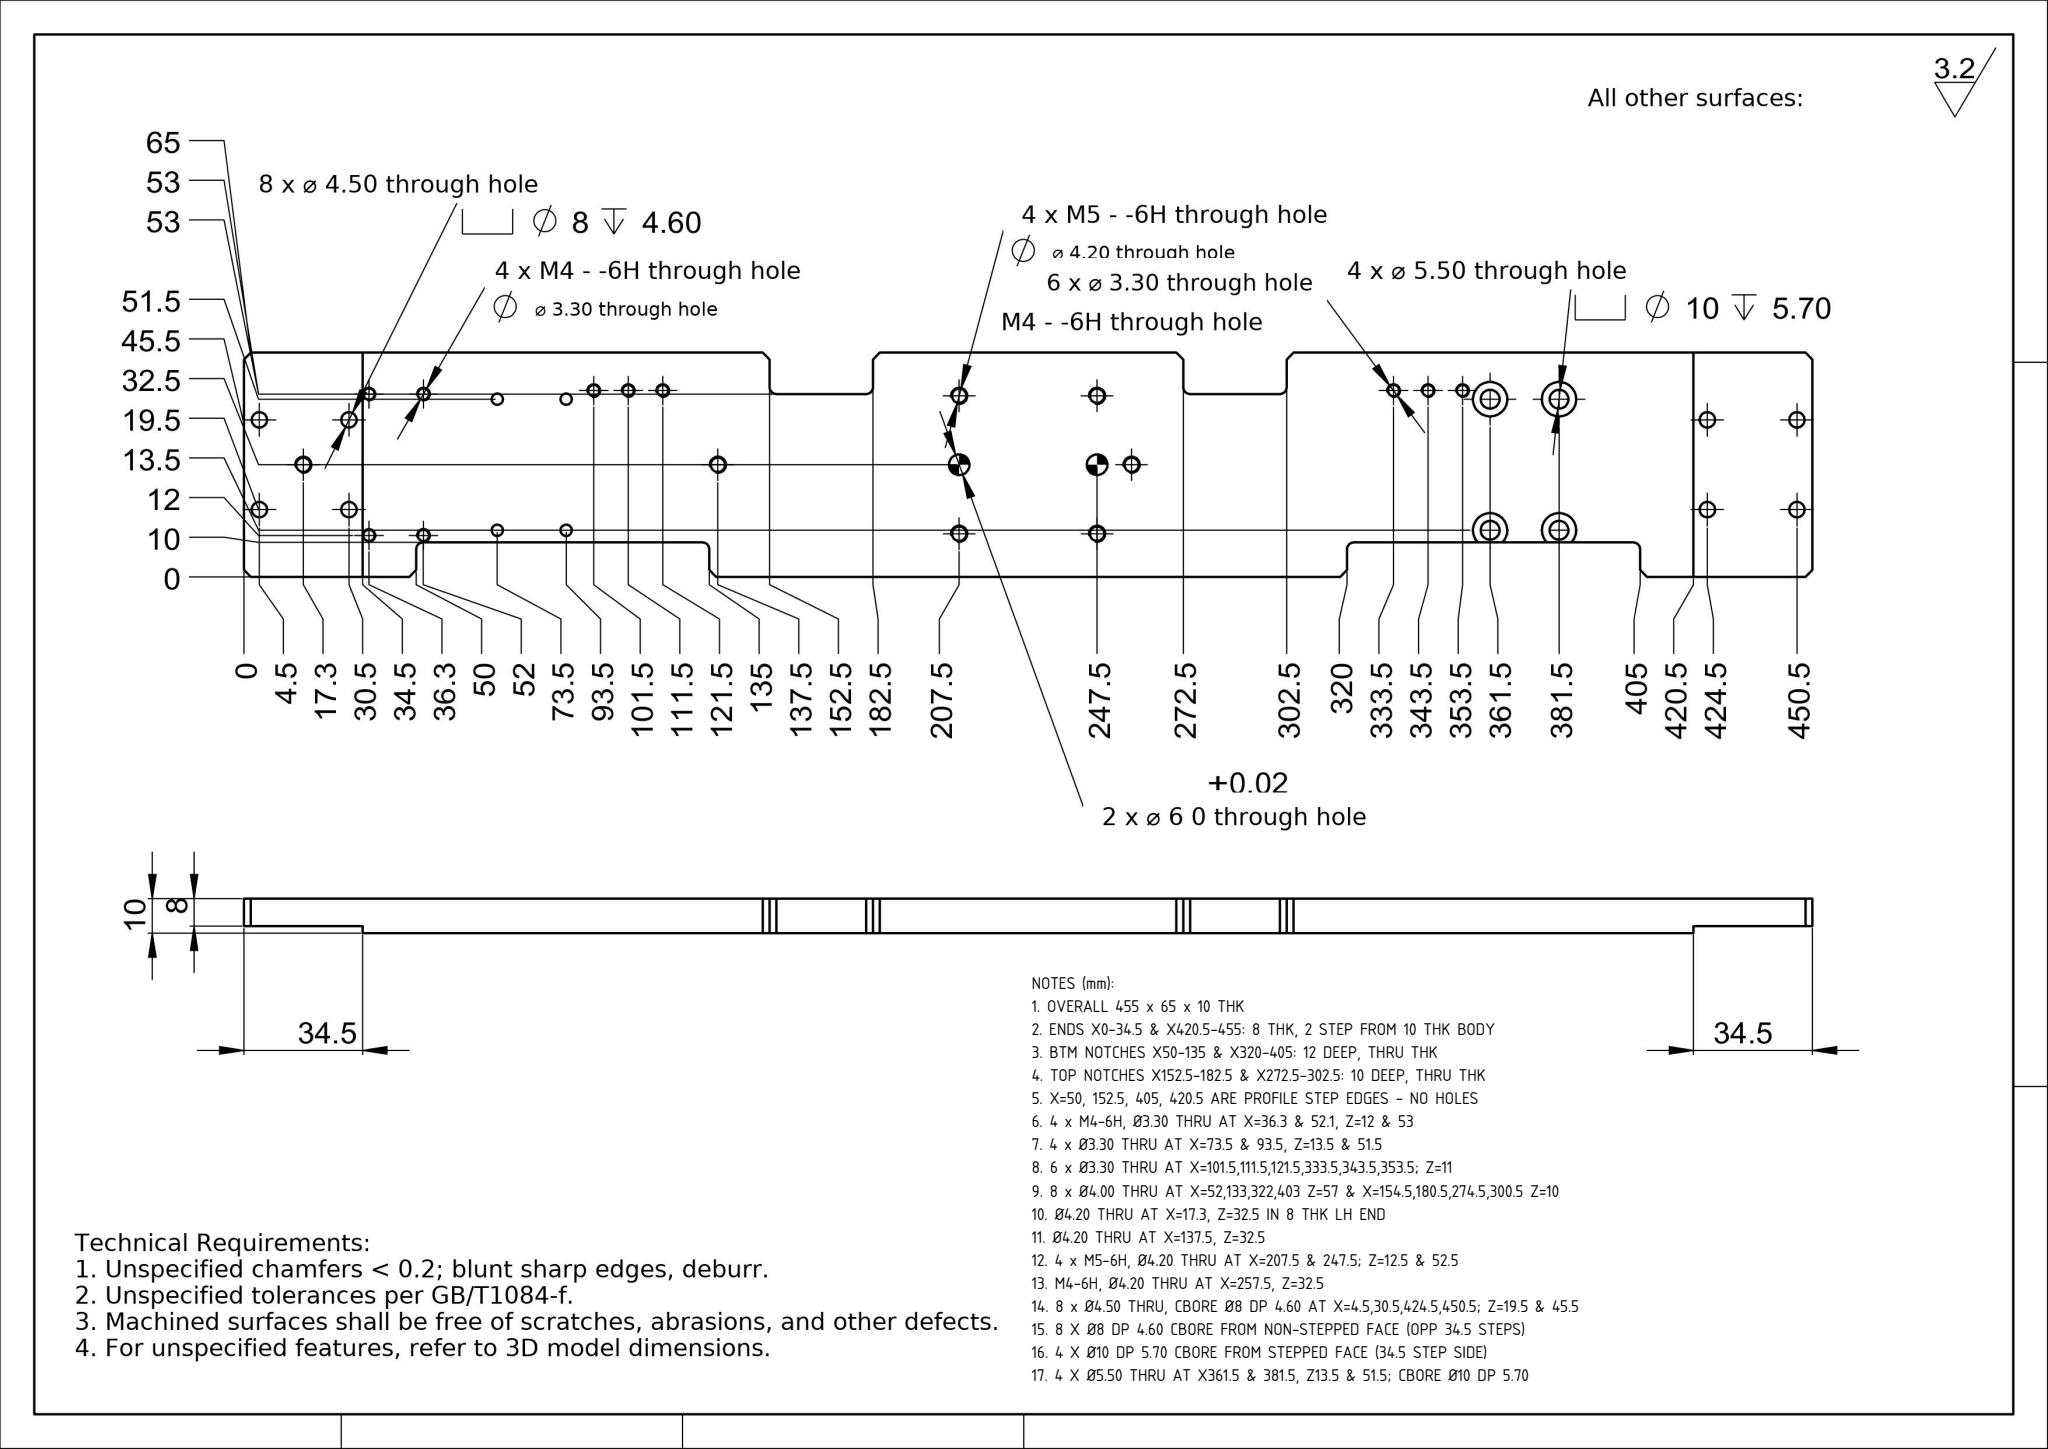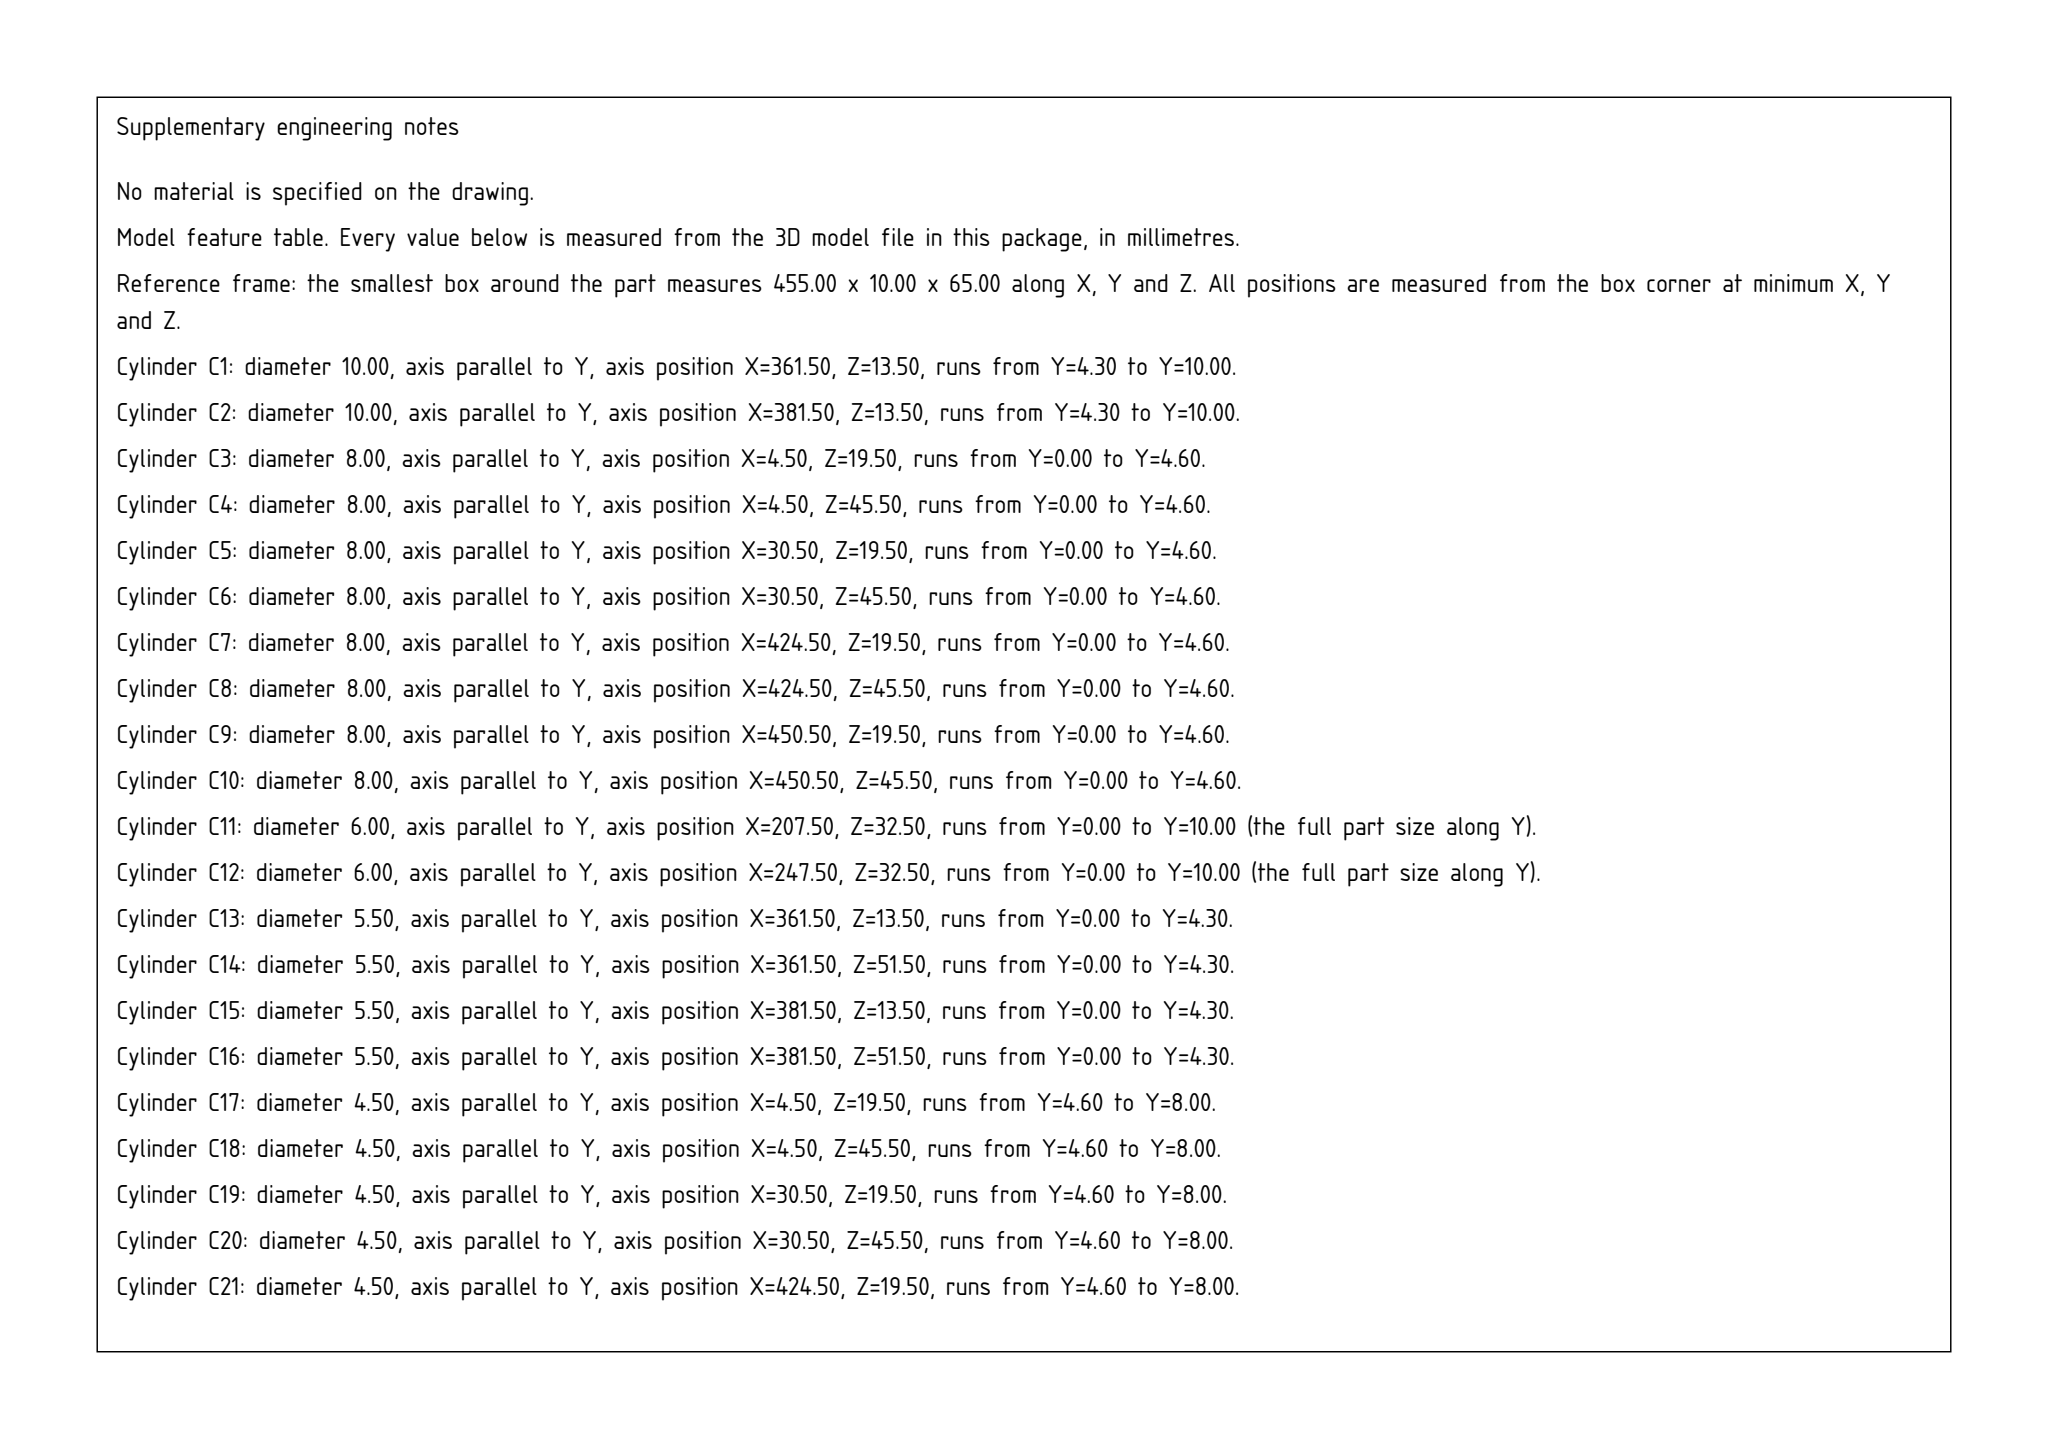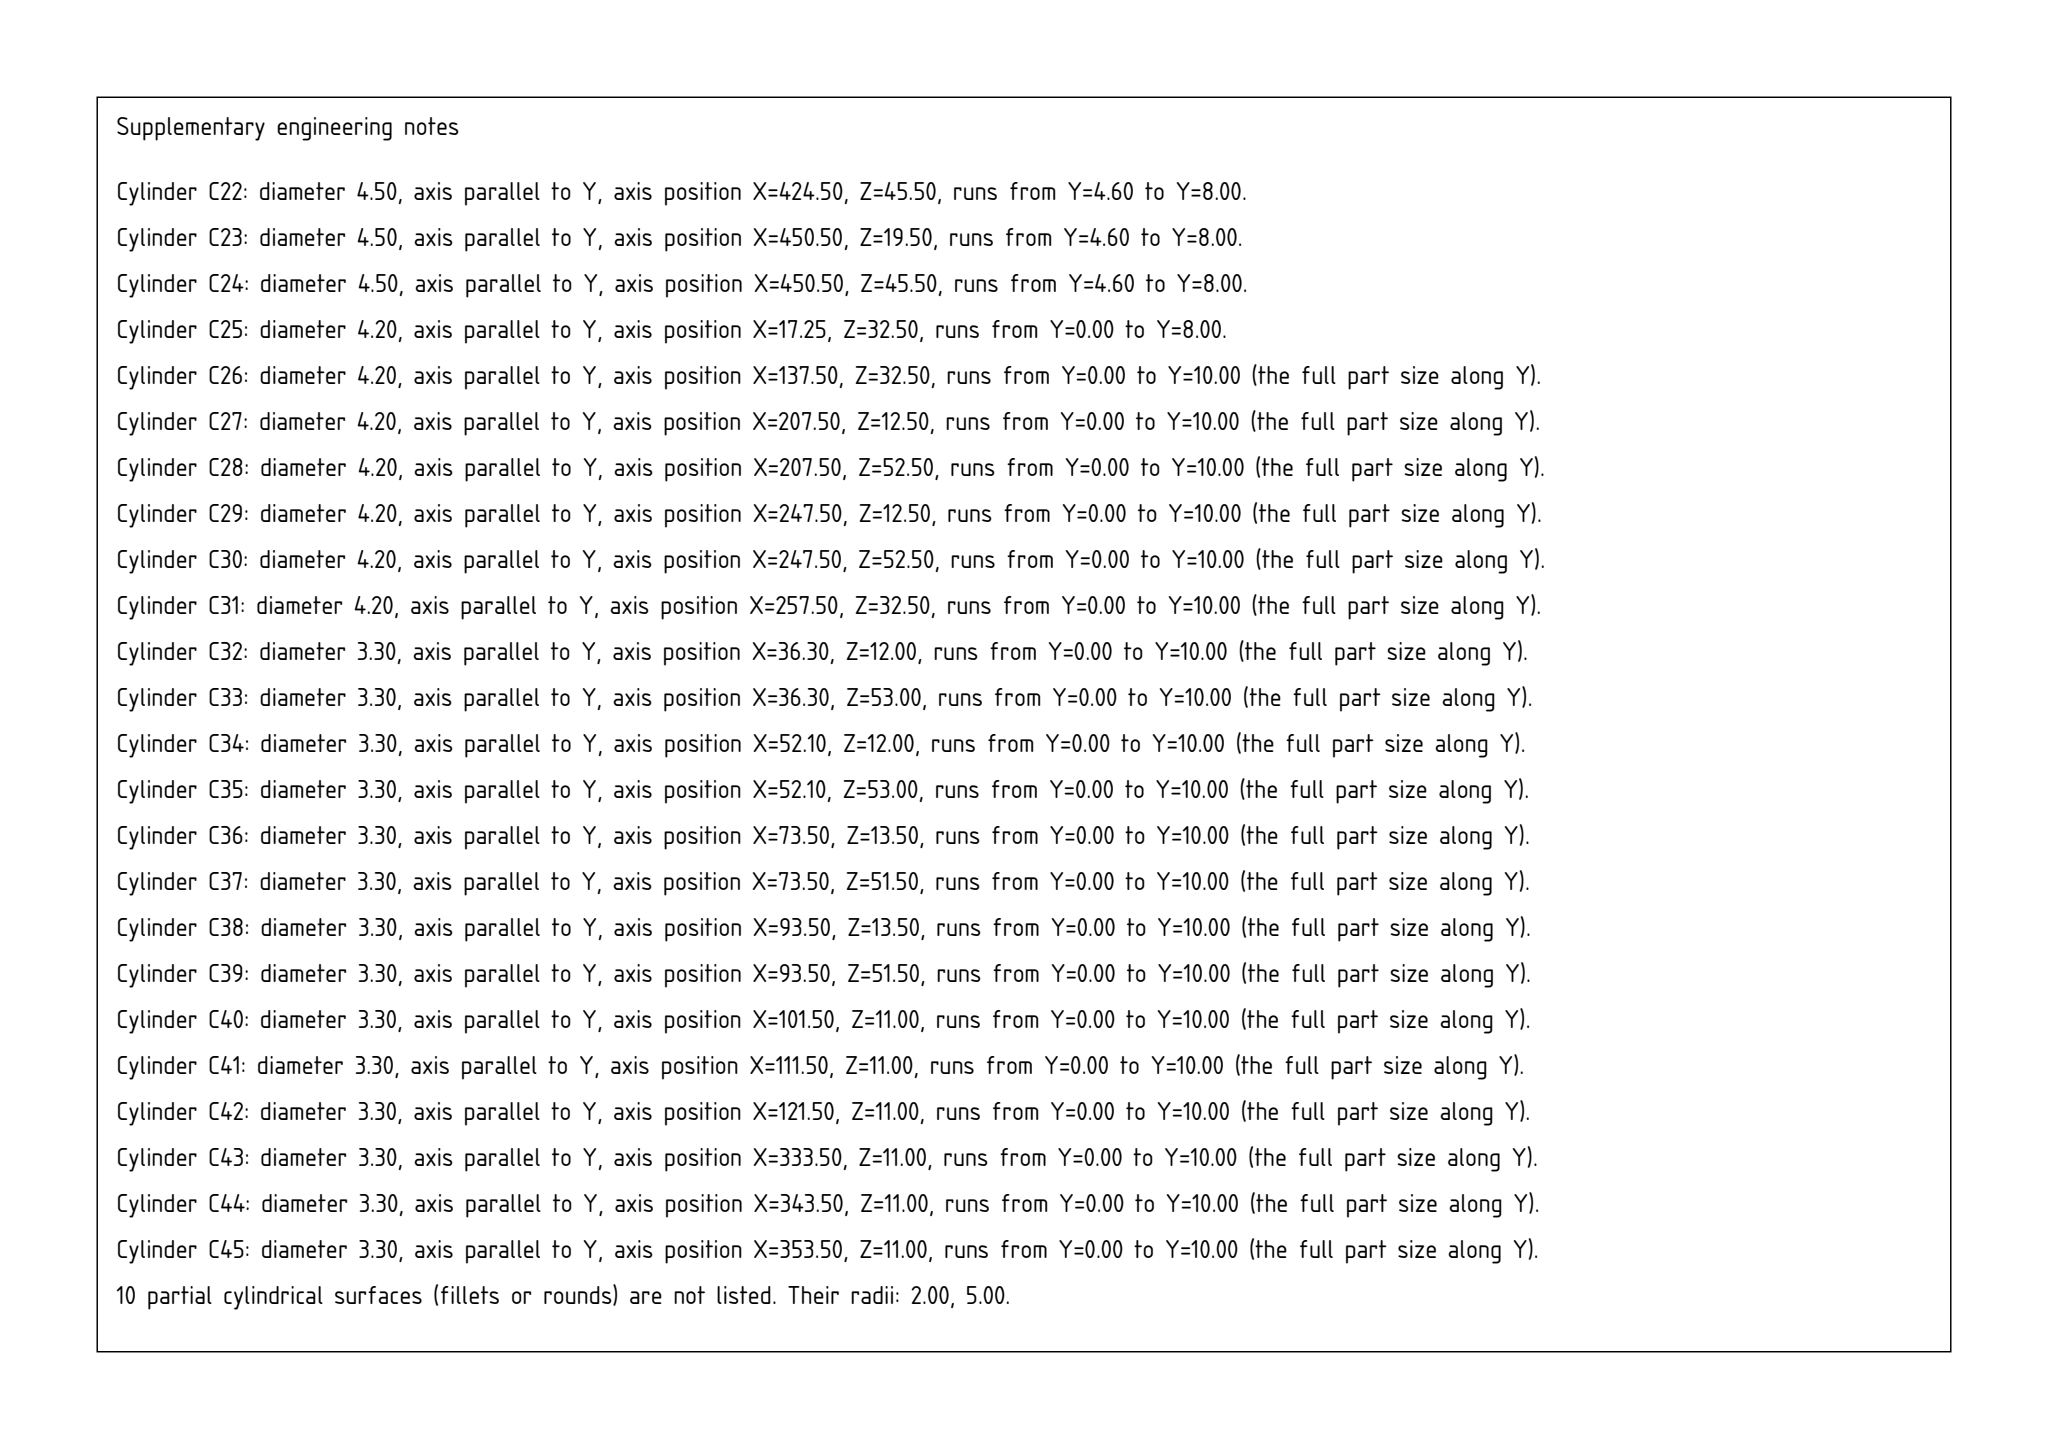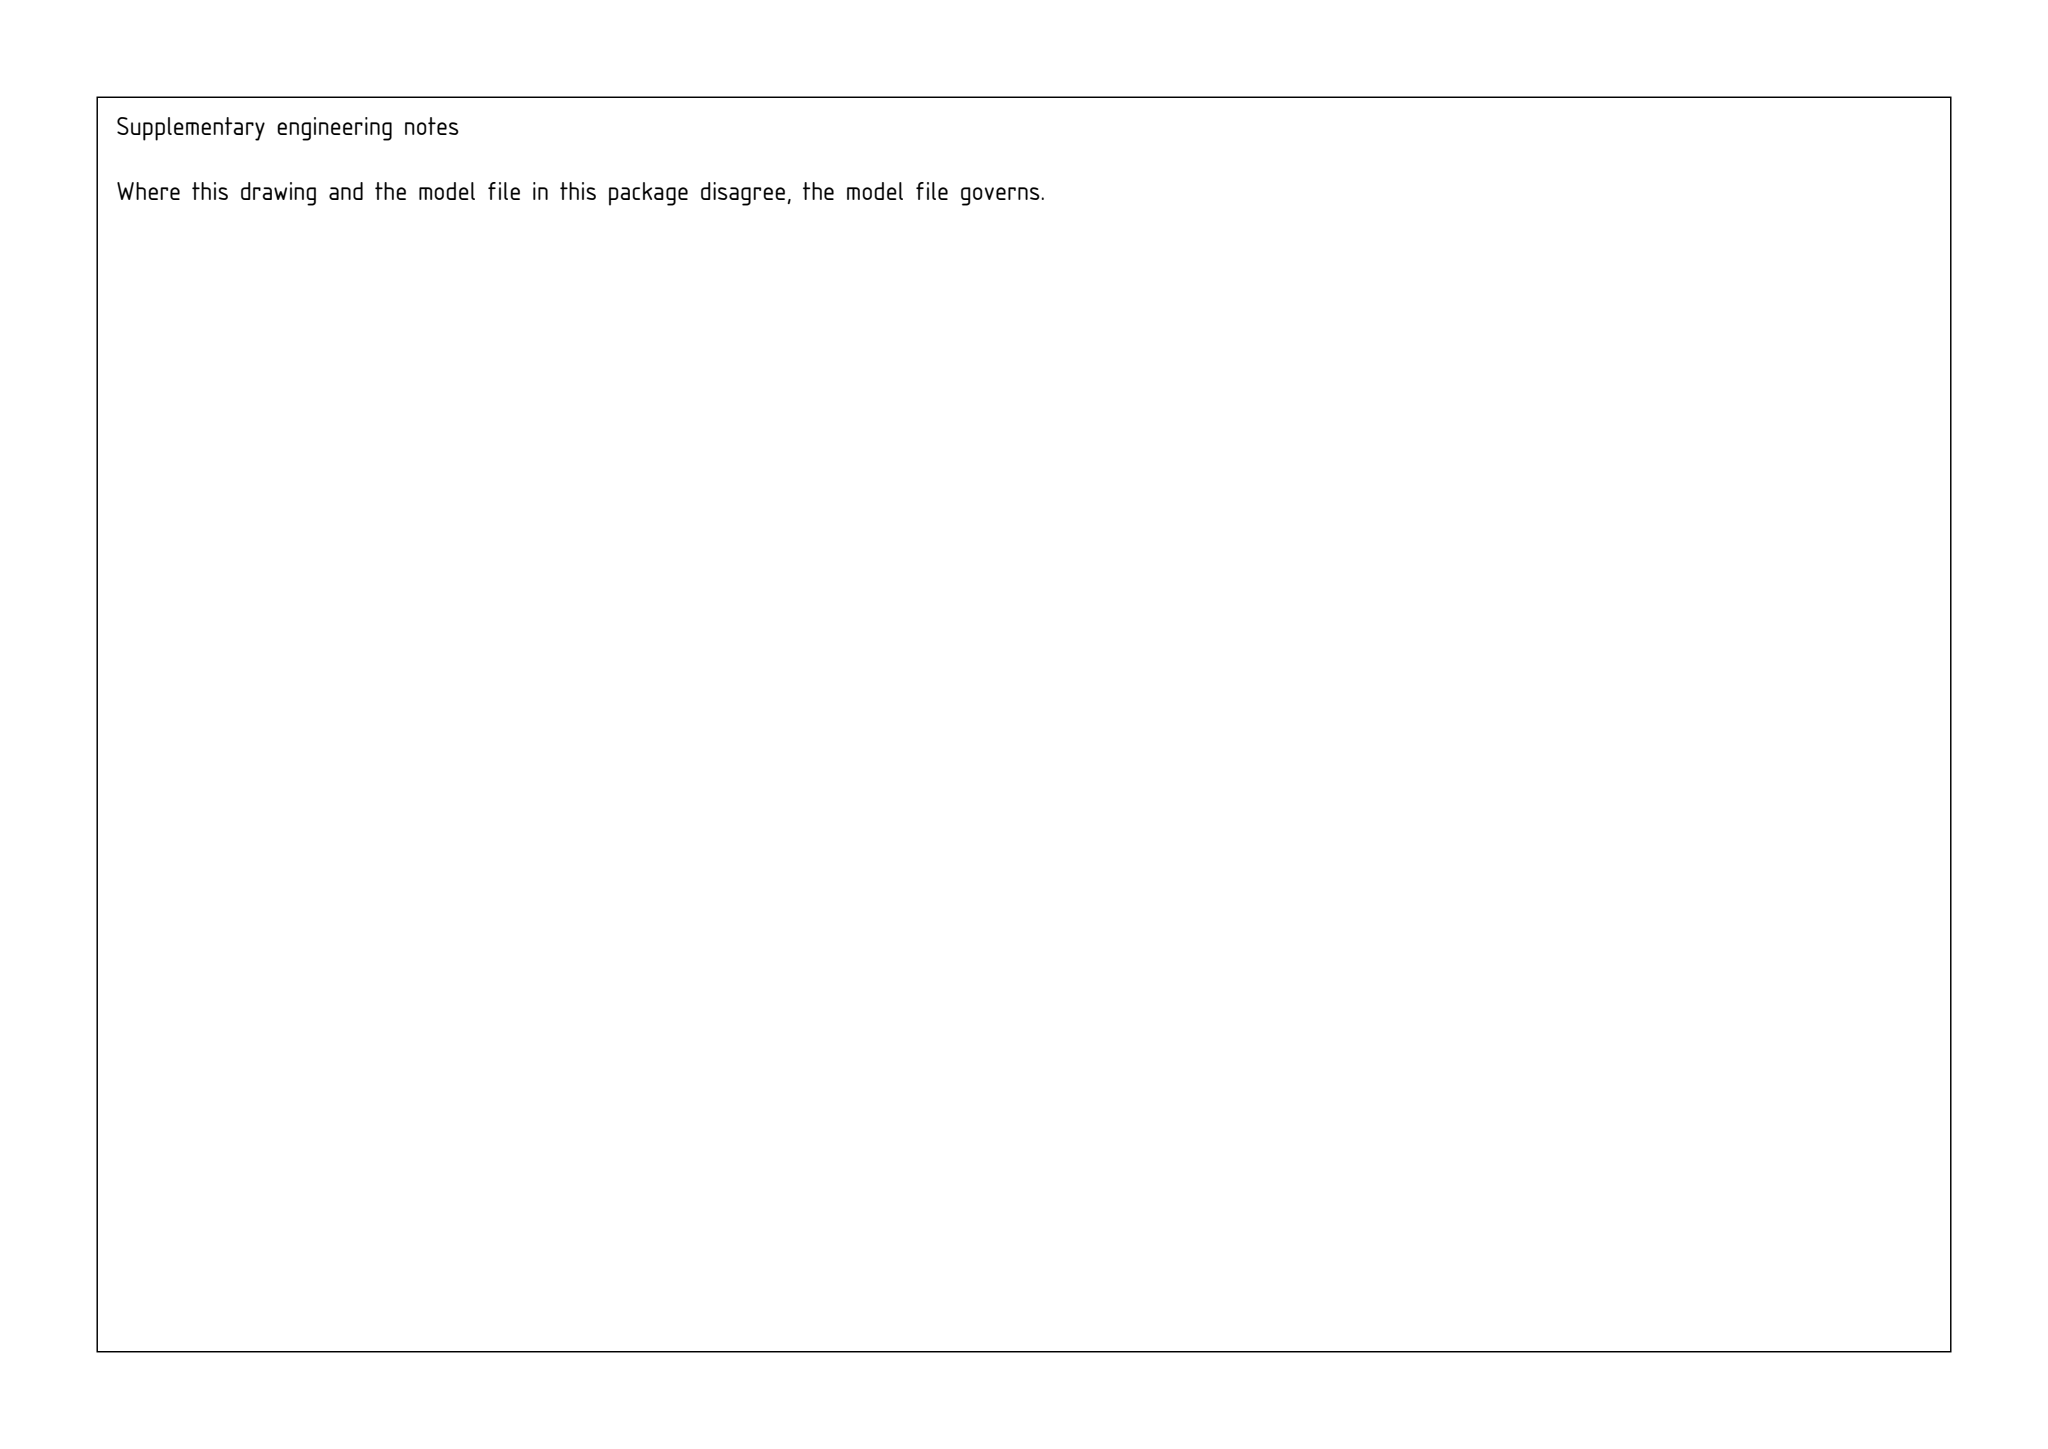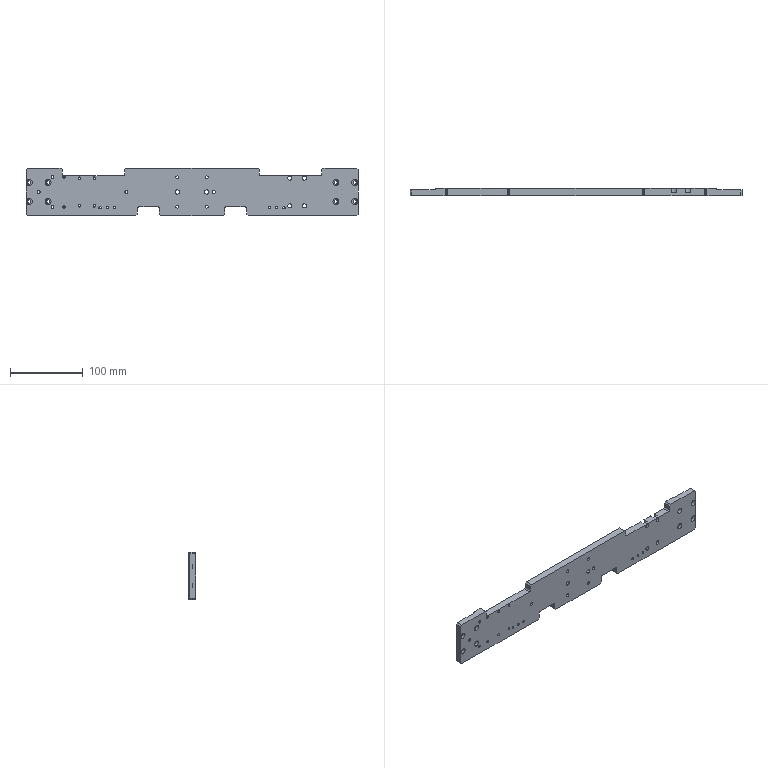Part | SolidWorks | mm | 1 solid | 150 faces | box 455 x 10 x 65 mm | volume 255322 mm3 | cylinder 100 | plane 50 | commonest cylinder face diameters 3.3 x28 8 x16 4.5 x16 4.2 x14 5.5 x8 4 x8 10 x6 6 x4
Drawing notes:
OVERALL 455 x 65 x 10 THK | from the solid: bbox_xyz 455.0 x 10.0 x 65.0
ENDS X0-34.5 & X420.5-455: 8 THK, 2 STEP FROM 10 THK BODY | from the solid: y planes 0, 8(2), 10(1); bbox y=10
BTM NOTCHES X50-135 & X320-405: 12 DEEP, THRU THK | from the solid: z planes 0(3) and 12(2); x planes 50,135,320,405
TOP NOTCHES X152.5-182.5 & X272.5-302.5: 10 DEEP, THRU THK | from the solid: z planes 65(3) and 55(2); x planes 152.5,182.5,272.5,302.5
X=50, 152.5, 405, 420.5 ARE PROFILE STEP EDGES - NO HOLES | from the solid: axis_planes x at 50,152.5,405,420.5; no cylinders at these x
4 x M4-6H, Ø3.30 THRU AT X=36.3 & 52.1, Z=12 & 53 | from the solid: cyl dia3.3 axis y at (36.3,12),(36.3,53),(52.1,12),(52.1,53), len 10
4 x Ø3.30 THRU AT X=73.5 & 93.5, Z=13.5 & 51.5 | from the solid: cyl dia3.3 axis y at (73.5,13.5),(73.5,51.5),(93.5,13.5),(93.5,51.5), len 10
6 x Ø3.30 THRU AT X=101.5,111.5,121.5,333.5,343.5,353.5; Z=11 | from the solid: cyl dia3.3 axis y at those x, z=11.0, len 10
8 x Ø4.00 THRU AT X=52,133,322,403 Z=57 & X=154.5,180.5,274.5,300.5 Z=10 | from the solid: cyl dia4.0 axis y, len 10, at listed x with z=57 and z=10
Ø4.20 THRU AT X=17.3, Z=32.5 IN 8 THK LH END | from the solid: cyl dia4.2 axis y at (17.25,32.5), len 8
Ø4.20 THRU AT X=137.5, Z=32.5 | from the solid: cyl dia4.2 axis y at (137.5,32.5), len 10
4 x M5-6H, Ø4.20 THRU AT X=207.5 & 247.5; Z=12.5 & 52.5 | from the solid: cyl dia4.2 axis y at (207.5/247.5, z=12.5/52.5), len 10
M4-6H, Ø4.20 THRU AT X=257.5, Z=32.5 | from the solid: cyl dia4.2 axis y at (257.5,32.5), len 10
8 x Ø4.50 THRU, CBORE Ø8 DP 4.60 AT X=4.5,30.5,424.5,450.5; Z=19.5 & 45.5 | from the solid: cyl dia4.5 len3.4 + dia8 len4.6 at x=4.5,30.5,424.5,450.5, z=19.5,45.5
8 X Ø8 DP 4.60 CBORE FROM NON-STEPPED FACE (OPP 34.5 STEPS) | from the solid: Ø8 CB depth 4.6 bottoms at y=4.6 plane; Ø4.5 thru 3.4 long spans y4.6-8.0 (8 THK end pads), so CB starts at y=0 face, i.e. the continuous face opposite the 34.5 steps (y=8 planes)
4 X Ø10 DP 5.70 CBORE FROM STEPPED FACE (34.5 STEP SIDE) | from the solid: Ø10 CB depth 5.7 bottoms at y=4.3 plane; Ø5.5 thru 4.3 long spans y0-4.3 in 10 THK web, so CB is cut from y=10 face = side containing the 34.5 steps
4 X Ø5.50 THRU AT X361.5 & 381.5, Z13.5 & 51.5; CBORE Ø10 DP 5.70 | from the solid: cylinders Ø5.5 at (361.5,13.5),(361.5,51.5),(381.5,13.5),(381.5,51.5) len 4.3, coaxial with Ø10 depth 5.7 counterbores at same 4 positions
build123d program:
from build123d import *

# Parameters (mm, degrees)
SKETCH1_W                                         = 455
SKETCH1_H                                         = 65
BOSS_EXTRUDE1_DEPTH                               = 5
HOLE_SIZE_ACCORDING_TO_TYPE_2_OF_HEXA_D           = 4.5
HOLE_SIZE_ACCORDING_TO_TYPE_2_OF_HEXA_CBORE_D     = 8
HOLE_SIZE_ACCORDING_TO_TYPE_2_OF_HEXA_CBORE_DEPTH = 4.6
HOLE_SIZE_ACCORDING_TO_TYPE_1_OF_HEXA_D           = 5.5
HOLE_SIZE_ACCORDING_TO_TYPE_1_OF_HEXA_CBORE_D     = 10
HOLE_SIZE_ACCORDING_TO_TYPE_1_OF_HEXA_CBORE_DEPTH = 5.7
M4_TAPPED_HOLE2_D                                 = 3.3
SKETCH11_W                                        = 34.5
SKETCH11_H                                        = 65
CUT_EXTRUDE2_DEPTH                                = 2
M5_TAPPED_HOLE3_D                                 = 4.2
M5_TAPPED_HOLE2_D                                 = 4.2
SKETCH16_W                                        = 85
SKETCH16_H                                        = 20
CUT_EXTRUDE3_DEPTH                                = 231.027
SIZE_MM_DOWEL_PIN_HOLE1_D                         = 6
CHAMFER1_SIZE                                     = 2
CHAMFER2_SIZE                                     = 2
FILLET1_R                                         = 2
M4_TAPPED_HOLE3_D                                 = 3.3
SKETCH19_W                                        = 30
SKETCH19_H                                        = 12
CUT_EXTRUDE4_DEPTH                                = 231.027
FILLET2_R                                         = 2
CHAMFER3_SIZE                                     = 2
M4_TAPPED_HOLE4_D                                 = 3.3
M4_TAPPED_HOLE4_DEPTH                             = 10.1
M4_TAPPED_HOLE4_TIP                               = 0.9914


with BuildPart() as part:
    # Sketch1 → Boss-Extrude1 (new, symmetric)
    with BuildSketch(Plane(origin=(0, 0, 0), x_dir=(1, 0, 0), z_dir=(0, 1, 0))):
        Rectangle(SKETCH1_W, SKETCH1_H)
    extrude(amount=BOSS_EXTRUDE1_DEPTH, both=True)

    # Hole Size _ according to_ Type 2 of Hexa (through all)
    with Locations(Plane(origin=(0, -5, 0), x_dir=(-1, 0, 0), z_dir=(0, -1, 0))):
        with Locations((-197, -13), (-223, 13), (-197, 13), (-223, -13), (223, -13), (197, 13), (223, 13), (197, -13)):
            CounterBoreHole(HOLE_SIZE_ACCORDING_TO_TYPE_2_OF_HEXA_D / 2, HOLE_SIZE_ACCORDING_TO_TYPE_2_OF_HEXA_CBORE_D / 2, HOLE_SIZE_ACCORDING_TO_TYPE_2_OF_HEXA_CBORE_DEPTH)

    # Hole Size _ according to_ Type 1 of Hexa (through all)
    with Locations(Plane(origin=(0, 5, 0), x_dir=(1, 0, 0), z_dir=(0, 1, 0))):
        with Locations((134, -19), (154, -19), (154, 19), (134, 19)):
            CounterBoreHole(HOLE_SIZE_ACCORDING_TO_TYPE_1_OF_HEXA_D / 2, HOLE_SIZE_ACCORDING_TO_TYPE_1_OF_HEXA_CBORE_D / 2, HOLE_SIZE_ACCORDING_TO_TYPE_1_OF_HEXA_CBORE_DEPTH)

    # M4 Tapped Hole2 (through all)
    with Locations(Plane(origin=(0, -5, 0), x_dir=(-1, 0, 0), z_dir=(0, -1, 0))):
        with Locations((175.4, 20.5), (191.2, 20.5), (175.4, -20.5), (191.2, -20.5)):
            Hole(M4_TAPPED_HOLE2_D / 2)

    # Sketch11 → Cut-Extrude2 (cut)
    with BuildSketch(Plane(origin=(0, 5, 0), x_dir=(1, 0, 0), z_dir=(0, 1, 0))):
        with Locations((210.25, 0)):
            Rectangle(SKETCH11_W, SKETCH11_H)
        with Locations((-210.25, 0)):
            Rectangle(SKETCH11_W, SKETCH11_H)
    extrude(amount=-CUT_EXTRUDE2_DEPTH, mode=Mode.SUBTRACT)

    # M5 Tapped Hole3 (through all)
    with Locations(Plane(origin=(0, 5, 0), x_dir=(1, 0, 0), z_dir=(0, 1, 0))):
        with Locations((-90, 0), (30, 0), (-210.25, 0)):
            Hole(M5_TAPPED_HOLE3_D / 2)

    # M5 Tapped Hole2 (through all)
    with Locations(Plane(origin=(0, 5, 0), x_dir=(1, 0, 0), z_dir=(0, 1, 0))):
        with Locations((-20, 20), (20, 20), (20, -20), (-20, -20)):
            Hole(M5_TAPPED_HOLE2_D / 2)

    # Sketch16 → Cut-Extrude3 (cut, through all)
    with BuildSketch(Plane(origin=(0, 5, 0), x_dir=(1, 0, 0), z_dir=(0, 1, 0))):
        with Locations((135, -32.5)):
            Rectangle(SKETCH16_W, SKETCH16_H)
        with Locations((-135, -32.5)):
            Rectangle(SKETCH16_W, SKETCH16_H)
    extrude(amount=-CUT_EXTRUDE3_DEPTH, mode=Mode.SUBTRACT)

    # Size mm Dowel Pin Hole1 (through all)
    with Locations(Plane(origin=(0, 5, 0), x_dir=(1, 0, 0), z_dir=(0, 1, 0))):
        with Locations((20, 0), (-20, 0)):
            Hole(SIZE_MM_DOWEL_PIN_HOLE1_D / 2)

    # Chamfer1
    chamfer1_edges = [part.edges().sort_by_distance(p)[0] for p in [
        (227.5, -1, 32.5),
        (227.5, -1, -32.5),
        (-227.5, -1, 32.5),
        (-227.5, -1, -32.5),
    ]]
    chamfer(chamfer1_edges, length=CHAMFER1_SIZE)

    # Chamfer2
    chamfer2_edges = [part.edges().sort_by_distance(p)[0] for p in [
        (177.5, 0, 32.5),
        (92.5, 0, 32.5),
        (-177.5, 0, 32.5),
        (-92.5, 0, 32.5),
    ]]
    chamfer(chamfer2_edges, length=CHAMFER2_SIZE)

    # Fillet1
    fillet1_edges = [part.edges().sort_by_distance(p)[0] for p in [
        (177.5, 0, 22.5),
        (92.5, 0, 22.5),
        (-92.5, 0, 22.5),
        (-177.5, 0, 22.5),
    ]]
    fillet(fillet1_edges, radius=FILLET1_R)

    # M4 Tapped Hole3 (through all)
    with Locations(Plane(origin=(0, 5, 0), x_dir=(1, 0, 0), z_dir=(0, 1, 0))):
        with Locations((106, 21.5), (116, 21.5), (126, 21.5)):
            m4_tapped_hole3 = Hole(M4_TAPPED_HOLE3_D / 2)

    # Sketch19 → Cut-Extrude4 (cut, through all)
    with BuildSketch(Plane(origin=(0, 5, 0), x_dir=(1, 0, 0), z_dir=(0, 1, 0))):
        with Locations((60, 26.5)):
            Rectangle(SKETCH19_W, SKETCH19_H)
    cut_extrude4 = extrude(amount=-CUT_EXTRUDE4_DEPTH, mode=Mode.SUBTRACT)

    # Mirror1: M4 Tapped Hole3, Cut-Extrude4 across plane
    add(m4_tapped_hole3.mirror(Plane(origin=(0, 0, 0), x_dir=(0, 0, 1), z_dir=(1, 0, 0))), mode=Mode.SUBTRACT)
    add(cut_extrude4.mirror(Plane(origin=(0, 0, 0), x_dir=(0, 0, 1), z_dir=(1, 0, 0))), mode=Mode.SUBTRACT)

    # Fillet2
    fillet2_edges = [part.edges().sort_by_distance(p)[0] for p in [
        (45, 0, -20.5),
        (75, 0, -20.5),
        (-45, 0, -20.5),
        (-75, 0, -20.5),
    ]]
    fillet(fillet2_edges, radius=FILLET2_R)

    # Chamfer3
    chamfer3_edges = [part.edges().sort_by_distance(p)[0] for p in [
        (45, 0, -32.5),
        (75, 0, -32.5),
        (-45, 0, -32.5),
        (-75, 0, -32.5),
    ]]
    chamfer(chamfer3_edges, length=CHAMFER3_SIZE)

    # M4 Tapped Hole4
    with Locations(Plane(origin=(0, -5, 0), x_dir=(-1, 0, 0), z_dir=(0, -1, 0))):
        with Locations((154, 19), (134, 19), (134, -19), (154, -19)):
            Hole(M4_TAPPED_HOLE4_D / 2, depth=M4_TAPPED_HOLE4_DEPTH)
            with Locations((0, 0, -(M4_TAPPED_HOLE4_DEPTH + M4_TAPPED_HOLE4_TIP / 2))):  # 118° drill point
                Cone(0, M4_TAPPED_HOLE4_D / 2, M4_TAPPED_HOLE4_TIP, mode=Mode.SUBTRACT)


solid = part.part